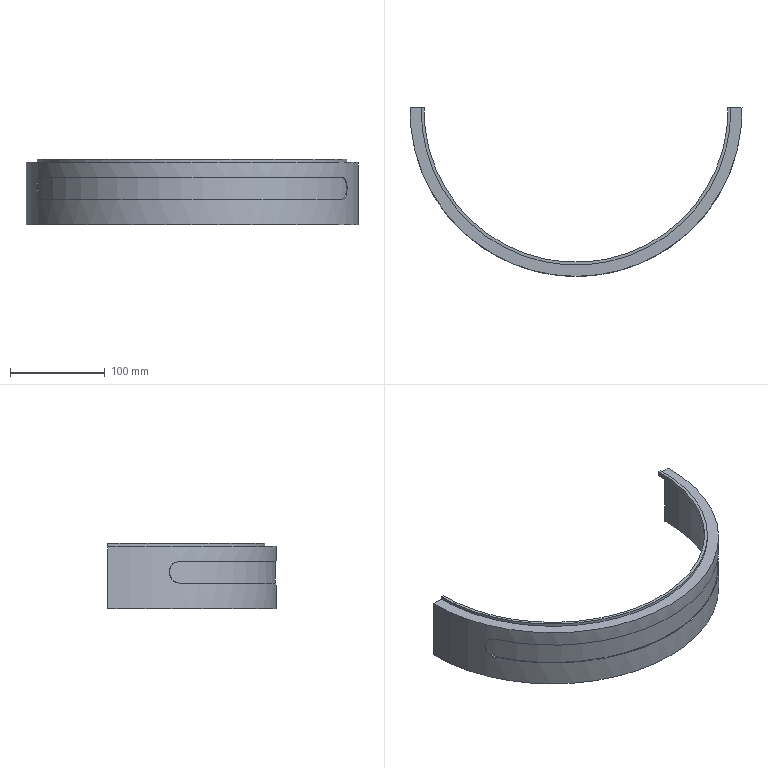Component | NX | FRONT_BAFFLE | 1 solid | 17 faces | volume 181677 mm3 | plane 10 | cylinder 7 | commonest cylinder face diameters 23 x2 349.761 x1 340 x1 320.161 x1 326.161 x1 347.755 x1